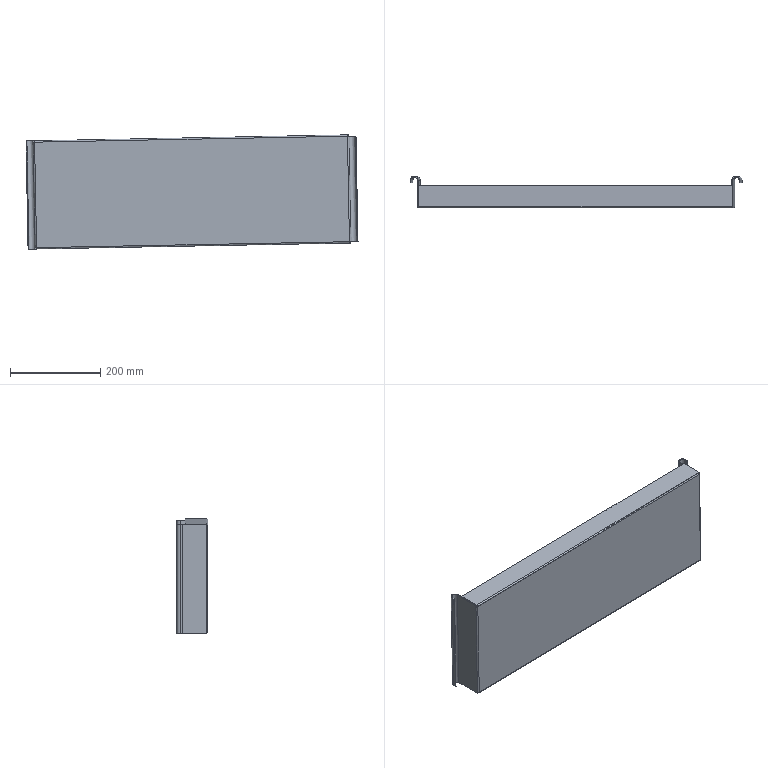Component | SolidWorks | 17DustCollectionHopper-3 | 1 solid | 58 faces | volume 551039 mm3 | plane 46 | cylinder 12 | commonest cylinder face diameters 6 x4 2 x4 18 x2 14 x2 | material A3 Steel